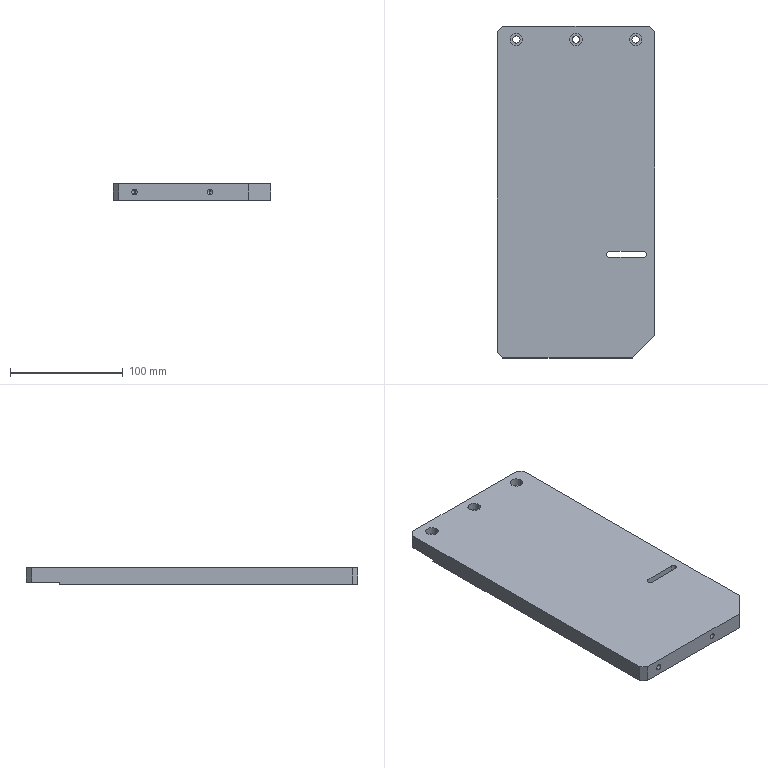Component | SolidWorks | XT-1-25-2-1 | 1 solid | 48 faces | box 140 x 295 x 15 mm | volume 601333 mm3 | cylinder 23 | plane 17 | cone 8 | commonest cylinder face diameters 11 x6 6.6 x6 4.2 x4 5 x4 5.3 x3
build123d program:
from build123d import *

# Parameters (mm, degrees)
SKETCH1_W                                            = 140
SKETCH1_H                                            = 350
BOSS_EXTRUDE1_DEPTH                                  = 15
SKETCH2_W                                            = 140
SKETCH2_H                                            = 30
CUT_EXTRUDE1_DEPTH                                   = 2
HOLE_SIZE_ACCORDING_TO_THE_TYPE_OF_HEXAG_D           = 6.6
HOLE_SIZE_ACCORDING_TO_THE_TYPE_OF_HEXAG_CBORE_D     = 11
HOLE_SIZE_ACCORDING_TO_THE_TYPE_OF_HEXAG_CBORE_DEPTH = 6.8
CUT_EXTRUDE4_DEPTH                                   = 190.077
CHAMFER2_SIZE                                        = 5
SKETCH16_W                                           = 150
SKETCH16_H                                           = 55
CUT_EXTRUDE5_DEPTH                                   = 190.077
M6_TAPPED_HOLE1_D                                    = 5
M6_TAPPED_HOLE1_DEPTH                                = 15
M6_TAPPED_HOLE1_TIP                                  = 1.502
CHAMFER3_SIZE                                        = 20
CHAMFER4_SIZE                                        = 5
M5_TAPPED_HOLE1_D                                    = 4.2
M5_TAPPED_HOLE1_DEPTH                                = 12.4
M5_TAPPED_HOLE1_TIP                                  = 1.262


with BuildPart() as part:
    # Sketch1 → Boss-Extrude1 (new body)
    with BuildSketch(Plane.XY):
        Rectangle(SKETCH1_W, SKETCH1_H)
    extrude(amount=BOSS_EXTRUDE1_DEPTH)

    # Sketch2 → Cut-Extrude1 (cut)
    with BuildSketch(Plane.XY.offset(15)):
        with Locations((0, 160)):
            Rectangle(SKETCH2_W, SKETCH2_H)
    extrude(amount=-CUT_EXTRUDE1_DEPTH, mode=Mode.SUBTRACT)

    # Hole Size according to the type of Hexag (through all)
    with Locations(Plane(origin=(0, 0, 0), x_dir=(-1, 0, 0), z_dir=(0, 0, -1))):
        with Locations((0, 163), (-53, 163), (53, 163)):
            CounterBoreHole(HOLE_SIZE_ACCORDING_TO_THE_TYPE_OF_HEXAG_D / 2, HOLE_SIZE_ACCORDING_TO_THE_TYPE_OF_HEXAG_CBORE_D / 2, HOLE_SIZE_ACCORDING_TO_THE_TYPE_OF_HEXAG_CBORE_DEPTH)

    # Sketch13 → Cut-Extrude4 (cut, through all)
    with BuildSketch(Plane(origin=(0, 0, 0), x_dir=(-1, 0, 0), z_dir=(0, 0, -1))):
        with BuildLine():
            Line((30, -25.35), (60, -25.35))
            ThreePointArc((60, -25.35), (62.65, -28), (60, -30.65))
            Line((60, -30.65), (30, -30.65))
            ThreePointArc((30, -30.65), (27.35, -28), (30, -25.35))
        make_face()
    extrude(amount=-CUT_EXTRUDE4_DEPTH, mode=Mode.SUBTRACT)

    # Chamfer2
    chamfer2_edges = [part.edges().sort_by_distance(p)[0] for p in [
        (-70, 175, 6.5),
        (70, 175, 6.5),
    ]]
    chamfer(chamfer2_edges, length=CHAMFER2_SIZE)

    # Sketch16 → Cut-Extrude5 (cut, through all)
    with BuildSketch(Plane.XY.offset(15)):
        with Locations((-5, -147.5)):
            Rectangle(SKETCH16_W, SKETCH16_H)
    extrude(amount=-CUT_EXTRUDE5_DEPTH, mode=Mode.SUBTRACT)

    # M6 Tapped Hole1
    with Locations(Plane(origin=(0, -120, 0), x_dir=(-1, 0, 0), z_dir=(0, -1, 0))):
        with Locations((-51, -7.5), (16, -7.5)):
            Hole(M6_TAPPED_HOLE1_D / 2, depth=M6_TAPPED_HOLE1_DEPTH)
            with Locations((0, 0, -(M6_TAPPED_HOLE1_DEPTH + M6_TAPPED_HOLE1_TIP / 2))):  # 118° drill point
                Cone(0, M6_TAPPED_HOLE1_D / 2, M6_TAPPED_HOLE1_TIP, mode=Mode.SUBTRACT)

    # Chamfer3
    chamfer3_edges = [part.edges().sort_by_distance(p)[0] for p in [
        (-70, -120, 7.5),
    ]]
    chamfer(chamfer3_edges, length=CHAMFER3_SIZE)

    # Chamfer4
    chamfer4_edges = [part.edges().sort_by_distance(p)[0] for p in [
        (70, -120, 7.5),
    ]]
    chamfer(chamfer4_edges, length=CHAMFER4_SIZE)

    # M5 Tapped Hole1
    with Locations(Plane.ZY.offset(70)):
        with Locations((7.5, -18), (7.5, -38)):
            Hole(M5_TAPPED_HOLE1_D / 2, depth=M5_TAPPED_HOLE1_DEPTH)
            with Locations((0, 0, -(M5_TAPPED_HOLE1_DEPTH + M5_TAPPED_HOLE1_TIP / 2))):  # 118° drill point
                Cone(0, M5_TAPPED_HOLE1_D / 2, M5_TAPPED_HOLE1_TIP, mode=Mode.SUBTRACT)


solid = part.part

# Placed as in the assembly
solid = solid.moved(Location((517.283, -90.615, 20.5), (-180, 0, 180)))